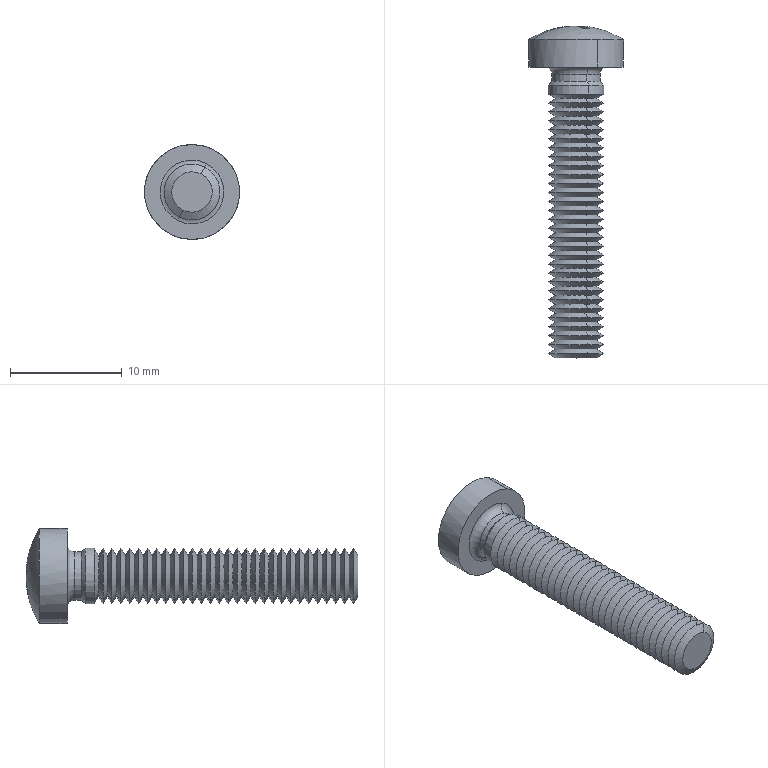Component | SolidWorks | GB_T818-2000PhillipsPanHeadScrewM5_25-4 | 1 solid | 144 faces | volume 558 mm3 | cone 120 | plane 14 | cylinder 6 | torus 2 | sphere 2 | commonest cylinder face diameters 5 x2 4.33 x2 8.5 x2